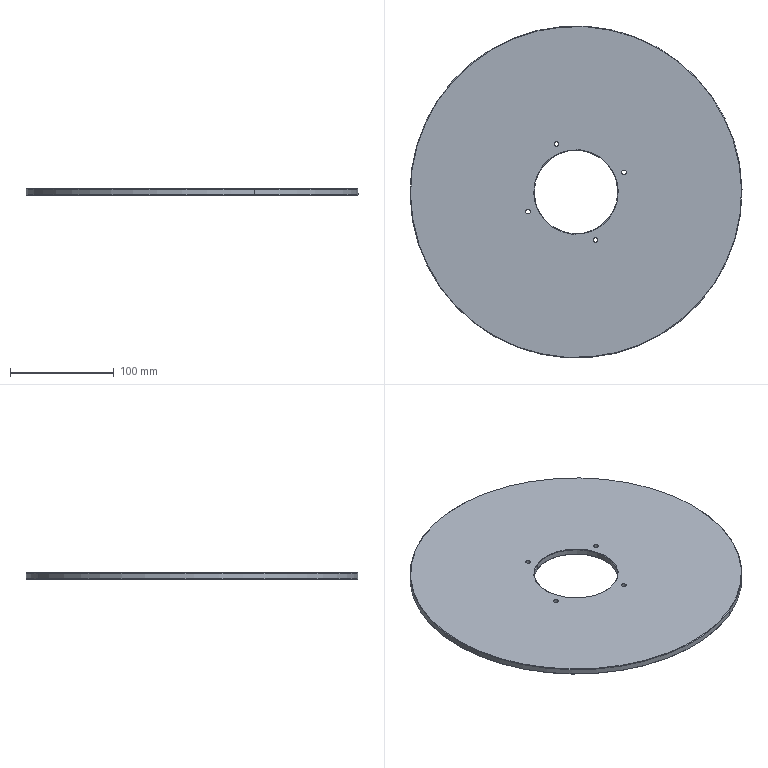Component | SolidWorks | 8TC-A17001-20-05Baffle2-1 | 1 solid | 30 faces | box 320 x 320 x 6 mm | volume 451128 mm3 | cone 16 | cylinder 12 | plane 2 | commonest cylinder face diameters 4.5 x8 80.5 x2 320 x2 | material Tempered Glass
STEP:
#1=COLOUR_RGB('',0.7922,0.8196,0.9333);
#2=FILL_AREA_STYLE_COLOUR('',#1);
#3=FILL_AREA_STYLE('',(#2));
#4=SURFACE_STYLE_FILL_AREA(#3);
#5=SURFACE_SIDE_STYLE('',(#4));
#6=SURFACE_STYLE_USAGE(.BOTH.,#5);
#7=PRESENTATION_STYLE_ASSIGNMENT((#6));
#8=CARTESIAN_POINT('',(26.486,13.716,9.39));
#9=VERTEX_POINT('',#8);
#10=CARTESIAN_POINT('',(31.233,2.089,9.39));
#11=VERTEX_POINT('',#10);
#12=CARTESIAN_POINT('',(28.859,7.902,9.39));
#13=DIRECTION('',(0.,-0.,1.));
#14=DIRECTION('',(-0.378,0.9258,0.));
#15=AXIS2_PLACEMENT_3D('',#12,#13,#14);
#16=CIRCLE('',#15,6.28);
#17=EDGE_CURVE('',#9,#11,#16,.T.);
#18=ORIENTED_EDGE('',*,*,#17,.F.);
#19=CARTESIAN_POINT('',(26.478,13.734,9.37));
#20=VERTEX_POINT('',#19);
#21=CARTESIAN_POINT('',(26.486,13.716,9.39));
#22=DIRECTION('',(-0.2673,0.6546,-0.7071));
#23=VECTOR('',#22,39.37);
#24=LINE('',#21,#23);
#25=EDGE_CURVE('',#9,#20,#24,.T.);
#26=ORIENTED_EDGE('',*,*,#25,.T.);
#27=CARTESIAN_POINT('',(31.241,2.071,9.37));
#28=VERTEX_POINT('',#27);
#29=CARTESIAN_POINT('',(28.859,7.902,9.37));
#30=DIRECTION('',(-0.,0.,-1.));
#31=DIRECTION('',(-0.378,0.9258,0.));
#32=AXIS2_PLACEMENT_3D('',#29,#30,#31);
#33=CIRCLE('',#32,6.299);
#34=EDGE_CURVE('',#28,#20,#33,.T.);
#35=ORIENTED_EDGE('',*,*,#34,.F.);
#36=CARTESIAN_POINT('',(31.233,2.089,9.39));
#37=DIRECTION('',(0.2673,-0.6546,-0.7071));
#38=VECTOR('',#37,39.37);
#39=LINE('',#36,#38);
#40=EDGE_CURVE('',#11,#28,#39,.T.);
#41=ORIENTED_EDGE('',*,*,#40,.F.);
#42=EDGE_LOOP('',(#18,#26,#35,#41));
#43=FACE_OUTER_BOUND('',#42,.T.);
#44=CARTESIAN_POINT('',(28.859,7.902,9.39));
#45=DIRECTION('',(-0.,0.,-1.));
#46=DIRECTION('',(0.378,-0.9258,-0.));
#47=AXIS2_PLACEMENT_3D('',#44,#45,#46);
#48=CONICAL_SURFACE('',#47,6.28,0.7854);
#49=ADVANCED_FACE('',(#43),#48,.T.);
#50=CARTESIAN_POINT('',(31.233,2.089,9.154));
#51=VERTEX_POINT('',#50);
#52=CARTESIAN_POINT('',(26.486,13.716,9.154));
#53=VERTEX_POINT('',#52);
#54=CARTESIAN_POINT('',(28.859,7.902,9.154));
#55=DIRECTION('',(-0.,0.,-1.));
#56=DIRECTION('',(-0.378,0.9258,0.));
#57=AXIS2_PLACEMENT_3D('',#54,#55,#56);
#58=CIRCLE('',#57,6.28);
#59=EDGE_CURVE('',#51,#53,#58,.T.);
#60=ORIENTED_EDGE('',*,*,#59,.F.);
#61=CARTESIAN_POINT('',(31.241,2.071,9.173));
#62=VERTEX_POINT('',#61);
#63=CARTESIAN_POINT('',(31.241,2.071,9.173));
#64=DIRECTION('',(0.2673,-0.6546,0.7071));
#65=VECTOR('',#64,39.37);
#66=LINE('',#63,#65);
#67=EDGE_CURVE('',#51,#62,#66,.T.);
#68=ORIENTED_EDGE('',*,*,#67,.T.);
#69=CARTESIAN_POINT('',(26.478,13.734,9.173));
#70=VERTEX_POINT('',#69);
#71=CARTESIAN_POINT('',(28.859,7.902,9.173));
#72=DIRECTION('',(0.,-0.,1.));
#73=DIRECTION('',(-0.378,0.9258,0.));
#74=AXIS2_PLACEMENT_3D('',#71,#72,#73);
#75=CIRCLE('',#74,6.299);
#76=EDGE_CURVE('',#70,#62,#75,.T.);
#77=ORIENTED_EDGE('',*,*,#76,.F.);
#78=CARTESIAN_POINT('',(26.478,13.734,9.173));
#79=DIRECTION('',(-0.2673,0.6546,0.7071));
#80=VECTOR('',#79,39.37);
#81=LINE('',#78,#80);
#82=EDGE_CURVE('',#53,#70,#81,.T.);
#83=ORIENTED_EDGE('',*,*,#82,.F.);
#84=EDGE_LOOP('',(#60,#68,#77,#83));
#85=FACE_OUTER_BOUND('',#84,.T.);
#86=CARTESIAN_POINT('',(28.859,7.902,9.173));
#87=DIRECTION('',(0.,-0.,1.));
#88=DIRECTION('',(-0.378,0.9258,0.));
#89=AXIS2_PLACEMENT_3D('',#86,#87,#88);
#90=CONICAL_SURFACE('',#89,6.299,0.7854);
#91=ADVANCED_FACE('',(#85),#90,.T.);
#92=CARTESIAN_POINT('',(29.458,6.435,9.37));
#93=VERTEX_POINT('',#92);
#94=CARTESIAN_POINT('',(28.26,9.369,9.37));
#95=VERTEX_POINT('',#94);
#96=CARTESIAN_POINT('',(28.859,7.902,9.37));
#97=DIRECTION('',(0.,-0.,1.));
#98=DIRECTION('',(-0.378,0.9258,0.));
#99=AXIS2_PLACEMENT_3D('',#96,#97,#98);
#100=CIRCLE('',#99,1.585);
#101=EDGE_CURVE('',#93,#95,#100,.T.);
#102=ORIENTED_EDGE('',*,*,#101,.F.);
#103=CARTESIAN_POINT('',(29.466,6.417,9.39));
#104=VERTEX_POINT('',#103);
#105=CARTESIAN_POINT('',(29.458,6.435,9.37));
#106=DIRECTION('',(0.2673,-0.6546,0.7071));
#107=VECTOR('',#106,39.37);
#108=LINE('',#105,#107);
#109=EDGE_CURVE('',#93,#104,#108,.T.);
#110=ORIENTED_EDGE('',*,*,#109,.T.);
#111=CARTESIAN_POINT('',(28.253,9.388,9.39));
#112=VERTEX_POINT('',#111);
#113=CARTESIAN_POINT('',(28.859,7.902,9.39));
#114=DIRECTION('',(-0.,0.,-1.));
#115=DIRECTION('',(-0.378,0.9258,0.));
#116=AXIS2_PLACEMENT_3D('',#113,#114,#115);
#117=CIRCLE('',#116,1.604);
#118=EDGE_CURVE('',#112,#104,#117,.T.);
#119=ORIENTED_EDGE('',*,*,#118,.F.);
#120=CARTESIAN_POINT('',(28.26,9.369,9.37));
#121=DIRECTION('',(-0.2673,0.6546,0.7071));
#122=VECTOR('',#121,39.37);
#123=LINE('',#120,#122);
#124=EDGE_CURVE('',#95,#112,#123,.T.);
#125=ORIENTED_EDGE('',*,*,#124,.F.);
#126=EDGE_LOOP('',(#102,#110,#119,#125));
#127=FACE_OUTER_BOUND('',#126,.T.);
#128=CARTESIAN_POINT('',(28.859,7.902,9.37));
#129=DIRECTION('',(0.,-0.,1.));
#130=DIRECTION('',(-0.378,0.9258,0.));
#131=AXIS2_PLACEMENT_3D('',#128,#129,#130);
#132=CONICAL_SURFACE('',#131,1.585,0.7854);
#133=ADVANCED_FACE('',(#127),#132,.F.);
#134=CARTESIAN_POINT('',(28.26,9.369,9.173));
#135=VERTEX_POINT('',#134);
#136=CARTESIAN_POINT('',(29.458,6.435,9.173));
#137=VERTEX_POINT('',#136);
#138=CARTESIAN_POINT('',(28.859,7.902,9.173));
#139=DIRECTION('',(-0.,0.,-1.));
#140=DIRECTION('',(-0.378,0.9258,0.));
#141=AXIS2_PLACEMENT_3D('',#138,#139,#140);
#142=CIRCLE('',#141,1.585);
#143=EDGE_CURVE('',#135,#137,#142,.T.);
#144=ORIENTED_EDGE('',*,*,#143,.F.);
#145=CARTESIAN_POINT('',(28.253,9.388,9.154));
#146=VERTEX_POINT('',#145);
#147=CARTESIAN_POINT('',(28.253,9.388,9.154));
#148=DIRECTION('',(-0.2673,0.6546,-0.7071));
#149=VECTOR('',#148,39.37);
#150=LINE('',#147,#149);
#151=EDGE_CURVE('',#135,#146,#150,.T.);
#152=ORIENTED_EDGE('',*,*,#151,.T.);
#153=CARTESIAN_POINT('',(29.466,6.417,9.154));
#154=VERTEX_POINT('',#153);
#155=CARTESIAN_POINT('',(28.859,7.902,9.154));
#156=DIRECTION('',(0.,-0.,1.));
#157=DIRECTION('',(-0.378,0.9258,0.));
#158=AXIS2_PLACEMENT_3D('',#155,#156,#157);
#159=CIRCLE('',#158,1.604);
#160=EDGE_CURVE('',#154,#146,#159,.T.);
#161=ORIENTED_EDGE('',*,*,#160,.F.);
#162=CARTESIAN_POINT('',(29.466,6.417,9.154));
#163=DIRECTION('',(0.2673,-0.6546,-0.7071));
#164=VECTOR('',#163,39.37);
#165=LINE('',#162,#164);
#166=EDGE_CURVE('',#137,#154,#165,.T.);
#167=ORIENTED_EDGE('',*,*,#166,.F.);
#168=EDGE_LOOP('',(#144,#152,#161,#167));
#169=FACE_OUTER_BOUND('',#168,.T.);
#170=CARTESIAN_POINT('',(28.859,7.902,9.154));
#171=DIRECTION('',(-0.,0.,-1.));
#172=DIRECTION('',(0.378,-0.9258,0.));
#173=AXIS2_PLACEMENT_3D('',#170,#171,#172);
#174=CONICAL_SURFACE('',#173,1.604,0.7854);
#175=ADVANCED_FACE('',(#169),#174,.F.);
#176=CARTESIAN_POINT('',(27.003,7.24,9.241));
#177=VERTEX_POINT('',#176);
#178=CARTESIAN_POINT('',(27.07,7.076,9.241));
#179=VERTEX_POINT('',#178);
#180=CARTESIAN_POINT('',(27.037,7.158,9.241));
#181=DIRECTION('',(-0.,0.,-1.));
#182=DIRECTION('',(0.378,-0.9258,0.));
#183=AXIS2_PLACEMENT_3D('',#180,#181,#182);
#184=CIRCLE('',#183,0.08858);
#185=EDGE_CURVE('',#177,#179,#184,.T.);
#186=ORIENTED_EDGE('',*,*,#185,.F.);
#187=CARTESIAN_POINT('',(26.97,7.322,9.154));
#188=VERTEX_POINT('',#187);
#189=CARTESIAN_POINT('',(26.97,7.322,9.154));
#190=DIRECTION('',(-0.2673,0.6546,-0.7071));
#191=VECTOR('',#190,39.37);
#192=LINE('',#189,#191);
#193=EDGE_CURVE('',#177,#188,#192,.T.);
#194=ORIENTED_EDGE('',*,*,#193,.T.);
#195=CARTESIAN_POINT('',(27.104,6.995,9.154));
#196=VERTEX_POINT('',#195);
#197=CARTESIAN_POINT('',(27.037,7.158,9.154));
#198=DIRECTION('',(-0.,0.,-1.));
#199=DIRECTION('',(0.378,-0.9258,0.));
#200=AXIS2_PLACEMENT_3D('',#197,#198,#199);
#201=CIRCLE('',#200,0.1764);
#202=EDGE_CURVE('',#188,#196,#201,.T.);
#203=ORIENTED_EDGE('',*,*,#202,.T.);
#204=CARTESIAN_POINT('',(27.104,6.995,9.154));
#205=DIRECTION('',(0.2673,-0.6546,-0.7071));
#206=VECTOR('',#205,39.37);
#207=LINE('',#204,#206);
#208=EDGE_CURVE('',#179,#196,#207,.T.);
#209=ORIENTED_EDGE('',*,*,#208,.F.);
#210=EDGE_LOOP('',(#186,#194,#203,#209));
#211=FACE_OUTER_BOUND('',#210,.T.);
#212=CARTESIAN_POINT('',(27.037,7.158,9.154));
#213=DIRECTION('',(-0.,0.,-1.));
#214=DIRECTION('',(0.378,-0.9258,0.));
#215=AXIS2_PLACEMENT_3D('',#212,#213,#214);
#216=CONICAL_SURFACE('',#215,0.1764,0.7854);
#217=ADVANCED_FACE('',(#211),#216,.F.);
#218=CARTESIAN_POINT('',(27.003,7.24,9.39));
#219=VERTEX_POINT('',#218);
#220=CARTESIAN_POINT('',(27.07,7.076,9.39));
#221=VERTEX_POINT('',#220);
#222=CARTESIAN_POINT('',(27.037,7.158,9.39));
#223=DIRECTION('',(-0.,0.,-1.));
#224=DIRECTION('',(0.378,-0.9258,0.));
#225=AXIS2_PLACEMENT_3D('',#222,#223,#224);
#226=CIRCLE('',#225,0.08858);
#227=EDGE_CURVE('',#219,#221,#226,.T.);
#228=ORIENTED_EDGE('',*,*,#227,.F.);
#229=CARTESIAN_POINT('',(27.003,7.24,9.154));
#230=DIRECTION('',(-0.,0.,-1.));
#231=VECTOR('',#230,39.37);
#232=LINE('',#229,#231);
#233=EDGE_CURVE('',#219,#177,#232,.T.);
#234=ORIENTED_EDGE('',*,*,#233,.T.);
#235=ORIENTED_EDGE('',*,*,#185,.T.);
#236=CARTESIAN_POINT('',(27.07,7.076,9.154));
#237=DIRECTION('',(-0.,0.,-1.));
#238=VECTOR('',#237,39.37);
#239=LINE('',#236,#238);
#240=EDGE_CURVE('',#221,#179,#239,.T.);
#241=ORIENTED_EDGE('',*,*,#240,.F.);
#242=EDGE_LOOP('',(#228,#234,#235,#241));
#243=FACE_OUTER_BOUND('',#242,.T.);
#244=CARTESIAN_POINT('',(27.037,7.158,9.154));
#245=DIRECTION('',(-0.,0.,-1.));
#246=DIRECTION('',(0.378,-0.9258,0.));
#247=AXIS2_PLACEMENT_3D('',#244,#245,#246);
#248=CYLINDRICAL_SURFACE('',#247,0.08858);
#249=ADVANCED_FACE('',(#243),#248,.F.);
#250=CARTESIAN_POINT('',(29.57,6.162,9.241));
#251=VERTEX_POINT('',#250);
#252=CARTESIAN_POINT('',(29.637,5.998,9.241));
#253=VERTEX_POINT('',#252);
#254=CARTESIAN_POINT('',(29.604,6.08,9.241));
#255=DIRECTION('',(-0.,0.,-1.));
#256=DIRECTION('',(0.378,-0.9258,0.));
#257=AXIS2_PLACEMENT_3D('',#254,#255,#256);
#258=CIRCLE('',#257,0.08858);
#259=EDGE_CURVE('',#251,#253,#258,.T.);
#260=ORIENTED_EDGE('',*,*,#259,.F.);
#261=CARTESIAN_POINT('',(29.537,6.243,9.154));
#262=VERTEX_POINT('',#261);
#263=CARTESIAN_POINT('',(29.537,6.243,9.154));
#264=DIRECTION('',(-0.2673,0.6546,-0.7071));
#265=VECTOR('',#264,39.37);
#266=LINE('',#263,#265);
#267=EDGE_CURVE('',#251,#262,#266,.T.);
#268=ORIENTED_EDGE('',*,*,#267,.T.);
#269=CARTESIAN_POINT('',(29.67,5.917,9.154));
#270=VERTEX_POINT('',#269);
#271=CARTESIAN_POINT('',(29.604,6.08,9.154));
#272=DIRECTION('',(-0.,0.,-1.));
#273=DIRECTION('',(0.378,-0.9258,0.));
#274=AXIS2_PLACEMENT_3D('',#271,#272,#273);
#275=CIRCLE('',#274,0.1764);
#276=EDGE_CURVE('',#262,#270,#275,.T.);
#277=ORIENTED_EDGE('',*,*,#276,.T.);
#278=CARTESIAN_POINT('',(29.67,5.917,9.154));
#279=DIRECTION('',(0.2673,-0.6546,-0.7071));
#280=VECTOR('',#279,39.37);
#281=LINE('',#278,#280);
#282=EDGE_CURVE('',#253,#270,#281,.T.);
#283=ORIENTED_EDGE('',*,*,#282,.F.);
#284=EDGE_LOOP('',(#260,#268,#277,#283));
#285=FACE_OUTER_BOUND('',#284,.T.);
#286=CARTESIAN_POINT('',(29.604,6.08,9.154));
#287=DIRECTION('',(-0.,0.,-1.));
#288=DIRECTION('',(0.378,-0.9258,0.));
#289=AXIS2_PLACEMENT_3D('',#286,#287,#288);
#290=CONICAL_SURFACE('',#289,0.1764,0.7854);
#291=ADVANCED_FACE('',(#285),#290,.F.);
#292=CARTESIAN_POINT('',(29.57,6.162,9.39));
#293=VERTEX_POINT('',#292);
#294=CARTESIAN_POINT('',(29.637,5.998,9.39));
#295=VERTEX_POINT('',#294);
#296=CARTESIAN_POINT('',(29.604,6.08,9.39));
#297=DIRECTION('',(-0.,0.,-1.));
#298=DIRECTION('',(0.378,-0.9258,0.));
#299=AXIS2_PLACEMENT_3D('',#296,#297,#298);
#300=CIRCLE('',#299,0.08858);
#301=EDGE_CURVE('',#293,#295,#300,.T.);
#302=ORIENTED_EDGE('',*,*,#301,.F.);
#303=CARTESIAN_POINT('',(29.57,6.162,9.154));
#304=DIRECTION('',(-0.,0.,-1.));
#305=VECTOR('',#304,39.37);
#306=LINE('',#303,#305);
#307=EDGE_CURVE('',#293,#251,#306,.T.);
#308=ORIENTED_EDGE('',*,*,#307,.T.);
#309=ORIENTED_EDGE('',*,*,#259,.T.);
#310=CARTESIAN_POINT('',(29.637,5.998,9.154));
#311=DIRECTION('',(-0.,0.,-1.));
#312=VECTOR('',#311,39.37);
#313=LINE('',#310,#312);
#314=EDGE_CURVE('',#295,#253,#313,.T.);
#315=ORIENTED_EDGE('',*,*,#314,.F.);
#316=EDGE_LOOP('',(#302,#308,#309,#315));
#317=FACE_OUTER_BOUND('',#316,.T.);
#318=CARTESIAN_POINT('',(29.604,6.08,9.154));
#319=DIRECTION('',(-0.,0.,-1.));
#320=DIRECTION('',(0.378,-0.9258,0.));
#321=AXIS2_PLACEMENT_3D('',#318,#319,#320);
#322=CYLINDRICAL_SURFACE('',#321,0.08858);
#323=ADVANCED_FACE('',(#317),#322,.F.);
#324=CARTESIAN_POINT('',(28.082,9.807,9.241));
#325=VERTEX_POINT('',#324);
#326=CARTESIAN_POINT('',(28.149,9.643,9.241));
#327=VERTEX_POINT('',#326);
#328=CARTESIAN_POINT('',(28.115,9.725,9.241));
#329=DIRECTION('',(-0.,0.,-1.));
#330=DIRECTION('',(0.378,-0.9258,0.));
#331=AXIS2_PLACEMENT_3D('',#328,#329,#330);
#332=CIRCLE('',#331,0.08858);
#333=EDGE_CURVE('',#325,#327,#332,.T.);
#334=ORIENTED_EDGE('',*,*,#333,.F.);
#335=CARTESIAN_POINT('',(28.049,9.888,9.154));
#336=VERTEX_POINT('',#335);
#337=CARTESIAN_POINT('',(28.049,9.888,9.154));
#338=DIRECTION('',(-0.2673,0.6546,-0.7071));
#339=VECTOR('',#338,39.37);
#340=LINE('',#337,#339);
#341=EDGE_CURVE('',#325,#336,#340,.T.);
#342=ORIENTED_EDGE('',*,*,#341,.T.);
#343=CARTESIAN_POINT('',(28.182,9.562,9.154));
#344=VERTEX_POINT('',#343);
#345=CARTESIAN_POINT('',(28.115,9.725,9.154));
#346=DIRECTION('',(-0.,0.,-1.));
#347=DIRECTION('',(0.378,-0.9258,0.));
#348=AXIS2_PLACEMENT_3D('',#345,#346,#347);
#349=CIRCLE('',#348,0.1764);
#350=EDGE_CURVE('',#336,#344,#349,.T.);
#351=ORIENTED_EDGE('',*,*,#350,.T.);
#352=CARTESIAN_POINT('',(28.182,9.562,9.154));
#353=DIRECTION('',(0.2673,-0.6546,-0.7071));
#354=VECTOR('',#353,39.37);
#355=LINE('',#352,#354);
#356=EDGE_CURVE('',#327,#344,#355,.T.);
#357=ORIENTED_EDGE('',*,*,#356,.F.);
#358=EDGE_LOOP('',(#334,#342,#351,#357));
#359=FACE_OUTER_BOUND('',#358,.T.);
#360=CARTESIAN_POINT('',(28.115,9.725,9.154));
#361=DIRECTION('',(-0.,0.,-1.));
#362=DIRECTION('',(0.378,-0.9258,0.));
#363=AXIS2_PLACEMENT_3D('',#360,#361,#362);
#364=CONICAL_SURFACE('',#363,0.1764,0.7854);
#365=ADVANCED_FACE('',(#359),#364,.F.);
#366=CARTESIAN_POINT('',(28.082,9.807,9.39));
#367=VERTEX_POINT('',#366);
#368=CARTESIAN_POINT('',(28.149,9.643,9.39));
#369=VERTEX_POINT('',#368);
#370=CARTESIAN_POINT('',(28.115,9.725,9.39));
#371=DIRECTION('',(-0.,0.,-1.));
#372=DIRECTION('',(0.378,-0.9258,0.));
#373=AXIS2_PLACEMENT_3D('',#370,#371,#372);
#374=CIRCLE('',#373,0.08858);
#375=EDGE_CURVE('',#367,#369,#374,.T.);
#376=ORIENTED_EDGE('',*,*,#375,.F.);
#377=CARTESIAN_POINT('',(28.082,9.807,9.154));
#378=DIRECTION('',(-0.,0.,-1.));
#379=VECTOR('',#378,39.37);
#380=LINE('',#377,#379);
#381=EDGE_CURVE('',#367,#325,#380,.T.);
#382=ORIENTED_EDGE('',*,*,#381,.T.);
#383=ORIENTED_EDGE('',*,*,#333,.T.);
#384=CARTESIAN_POINT('',(28.149,9.643,9.154));
#385=DIRECTION('',(-0.,0.,-1.));
#386=VECTOR('',#385,39.37);
#387=LINE('',#384,#386);
#388=EDGE_CURVE('',#369,#327,#387,.T.);
#389=ORIENTED_EDGE('',*,*,#388,.F.);
#390=EDGE_LOOP('',(#376,#382,#383,#389));
#391=FACE_OUTER_BOUND('',#390,.T.);
#392=CARTESIAN_POINT('',(28.115,9.725,9.154));
#393=DIRECTION('',(-0.,0.,-1.));
#394=DIRECTION('',(0.378,-0.9258,0.));
#395=AXIS2_PLACEMENT_3D('',#392,#393,#394);
#396=CYLINDRICAL_SURFACE('',#395,0.08858);
#397=ADVANCED_FACE('',(#391),#396,.F.);
#398=CARTESIAN_POINT('',(30.648,8.729,9.241));
#399=VERTEX_POINT('',#398);
#400=CARTESIAN_POINT('',(30.715,8.565,9.241));
#401=VERTEX_POINT('',#400);
#402=CARTESIAN_POINT('',(30.682,8.647,9.241));
#403=DIRECTION('',(-0.,0.,-1.));
#404=DIRECTION('',(0.378,-0.9258,0.));
#405=AXIS2_PLACEMENT_3D('',#402,#403,#404);
#406=CIRCLE('',#405,0.08858);
#407=EDGE_CURVE('',#399,#401,#406,.T.);
#408=ORIENTED_EDGE('',*,*,#407,.F.);
#409=CARTESIAN_POINT('',(30.615,8.81,9.154));
#410=VERTEX_POINT('',#409);
#411=CARTESIAN_POINT('',(30.615,8.81,9.154));
#412=DIRECTION('',(-0.2673,0.6546,-0.7071));
#413=VECTOR('',#412,39.37);
#414=LINE('',#411,#413);
#415=EDGE_CURVE('',#399,#410,#414,.T.);
#416=ORIENTED_EDGE('',*,*,#415,.T.);
#417=CARTESIAN_POINT('',(30.749,8.483,9.154));
#418=VERTEX_POINT('',#417);
#419=CARTESIAN_POINT('',(30.682,8.647,9.154));
#420=DIRECTION('',(-0.,0.,-1.));
#421=DIRECTION('',(0.378,-0.9258,0.));
#422=AXIS2_PLACEMENT_3D('',#419,#420,#421);
#423=CIRCLE('',#422,0.1764);
#424=EDGE_CURVE('',#410,#418,#423,.T.);
#425=ORIENTED_EDGE('',*,*,#424,.T.);
#426=CARTESIAN_POINT('',(30.749,8.483,9.154));
#427=DIRECTION('',(0.2673,-0.6546,-0.7071));
#428=VECTOR('',#427,39.37);
#429=LINE('',#426,#428);
#430=EDGE_CURVE('',#401,#418,#429,.T.);
#431=ORIENTED_EDGE('',*,*,#430,.F.);
#432=EDGE_LOOP('',(#408,#416,#425,#431));
#433=FACE_OUTER_BOUND('',#432,.T.);
#434=CARTESIAN_POINT('',(30.682,8.647,9.154));
#435=DIRECTION('',(-0.,0.,-1.));
#436=DIRECTION('',(0.378,-0.9258,0.));
#437=AXIS2_PLACEMENT_3D('',#434,#435,#436);
#438=CONICAL_SURFACE('',#437,0.1764,0.7854);
#439=ADVANCED_FACE('',(#433),#438,.F.);
#440=CARTESIAN_POINT('',(30.648,8.729,9.39));
#441=VERTEX_POINT('',#440);
#442=CARTESIAN_POINT('',(30.715,8.565,9.39));
#443=VERTEX_POINT('',#442);
#444=CARTESIAN_POINT('',(30.682,8.647,9.39));
#445=DIRECTION('',(-0.,0.,-1.));
#446=DIRECTION('',(0.378,-0.9258,0.));
#447=AXIS2_PLACEMENT_3D('',#444,#445,#446);
#448=CIRCLE('',#447,0.08858);
#449=EDGE_CURVE('',#441,#443,#448,.T.);
#450=ORIENTED_EDGE('',*,*,#449,.F.);
#451=CARTESIAN_POINT('',(30.648,8.729,9.154));
#452=DIRECTION('',(-0.,0.,-1.));
#453=VECTOR('',#452,39.37);
#454=LINE('',#451,#453);
#455=EDGE_CURVE('',#441,#399,#454,.T.);
#456=ORIENTED_EDGE('',*,*,#455,.T.);
#457=ORIENTED_EDGE('',*,*,#407,.T.);
#458=CARTESIAN_POINT('',(30.715,8.565,9.154));
#459=DIRECTION('',(-0.,0.,-1.));
#460=VECTOR('',#459,39.37);
#461=LINE('',#458,#460);
#462=EDGE_CURVE('',#443,#401,#461,.T.);
#463=ORIENTED_EDGE('',*,*,#462,.F.);
#464=EDGE_LOOP('',(#450,#456,#457,#463));
#465=FACE_OUTER_BOUND('',#464,.T.);
#466=CARTESIAN_POINT('',(30.682,8.647,9.154));
#467=DIRECTION('',(-0.,0.,-1.));
#468=DIRECTION('',(0.378,-0.9258,0.));
#469=AXIS2_PLACEMENT_3D('',#466,#467,#468);
#470=CYLINDRICAL_SURFACE('',#469,0.08858);
#471=ADVANCED_FACE('',(#465),#470,.F.);
#472=ORIENTED_EDGE('',*,*,#101,.T.);
#473=CARTESIAN_POINT('',(28.26,9.369,9.39));
#474=DIRECTION('',(-0.,0.,-1.));
#475=VECTOR('',#474,39.37);
#476=LINE('',#473,#475);
#477=EDGE_CURVE('',#95,#135,#476,.T.);
#478=ORIENTED_EDGE('',*,*,#477,.T.);
#479=ORIENTED_EDGE('',*,*,#143,.T.);
#480=CARTESIAN_POINT('',(29.458,6.435,9.39));
#481=DIRECTION('',(-0.,0.,-1.));
#482=VECTOR('',#481,39.37);
#483=LINE('',#480,#482);
#484=EDGE_CURVE('',#93,#137,#483,.T.);
#485=ORIENTED_EDGE('',*,*,#484,.F.);
#486=EDGE_LOOP('',(#472,#478,#479,#485));
#487=FACE_OUTER_BOUND('',#486,.T.);
#488=CARTESIAN_POINT('',(28.859,7.902,9.39));
#489=DIRECTION('',(-0.,0.,-1.));
#490=DIRECTION('',(0.378,-0.9258,0.));
#491=AXIS2_PLACEMENT_3D('',#488,#489,#490);
#492=CYLINDRICAL_SURFACE('',#491,1.585);
#493=ADVANCED_FACE('',(#487),#492,.F.);
#494=ORIENTED_EDGE('',*,*,#34,.T.);
#495=CARTESIAN_POINT('',(26.478,13.734,9.39));
#496=DIRECTION('',(-0.,0.,-1.));
#497=VECTOR('',#496,39.37);
#498=LINE('',#495,#497);
#499=EDGE_CURVE('',#20,#70,#498,.T.);
#500=ORIENTED_EDGE('',*,*,#499,.T.);
#501=ORIENTED_EDGE('',*,*,#76,.T.);
#502=CARTESIAN_POINT('',(31.241,2.071,9.39));
#503=DIRECTION('',(-0.,0.,-1.));
#504=VECTOR('',#503,39.37);
#505=LINE('',#502,#504);
#506=EDGE_CURVE('',#28,#62,#505,.T.);
#507=ORIENTED_EDGE('',*,*,#506,.F.);
#508=EDGE_LOOP('',(#494,#500,#501,#507));
#509=FACE_OUTER_BOUND('',#508,.T.);
#510=CARTESIAN_POINT('',(28.859,7.902,9.39));
#511=DIRECTION('',(-0.,0.,-1.));
#512=DIRECTION('',(0.378,-0.9258,-0.));
#513=AXIS2_PLACEMENT_3D('',#510,#511,#512);
#514=CYLINDRICAL_SURFACE('',#513,6.299);
#515=ADVANCED_FACE('',(#509),#514,.T.);
#516=ORIENTED_EDGE('',*,*,#118,.T.);
#517=CARTESIAN_POINT('',(28.859,7.902,9.39));
#518=DIRECTION('',(-0.,0.,-1.));
#519=DIRECTION('',(-0.378,0.9258,0.));
#520=AXIS2_PLACEMENT_3D('',#517,#518,#519);
#521=CIRCLE('',#520,1.604);
#522=EDGE_CURVE('',#104,#112,#521,.T.);
#523=ORIENTED_EDGE('',*,*,#522,.T.);
#524=EDGE_LOOP('',(#516,#523));
#525=FACE_BOUND('',#524,.T.);
#526=CARTESIAN_POINT('',(28.859,7.902,9.39));
#527=DIRECTION('',(0.,-0.,1.));
#528=DIRECTION('',(-0.378,0.9258,0.));
#529=AXIS2_PLACEMENT_3D('',#526,#527,#528);
#530=CIRCLE('',#529,6.28);
#531=EDGE_CURVE('',#11,#9,#530,.T.);
#532=ORIENTED_EDGE('',*,*,#531,.T.);
#533=ORIENTED_EDGE('',*,*,#17,.T.);
#534=EDGE_LOOP('',(#532,#533));
#535=FACE_OUTER_BOUND('',#534,.T.);
#536=CARTESIAN_POINT('',(27.037,7.158,9.39));
#537=DIRECTION('',(-0.,0.,-1.));
#538=DIRECTION('',(0.378,-0.9258,0.));
#539=AXIS2_PLACEMENT_3D('',#536,#537,#538);
#540=CIRCLE('',#539,0.08858);
#541=EDGE_CURVE('',#221,#219,#540,.T.);
#542=ORIENTED_EDGE('',*,*,#541,.T.);
#543=ORIENTED_EDGE('',*,*,#227,.T.);
#544=EDGE_LOOP('',(#542,#543));
#545=FACE_BOUND('',#544,.T.);
#546=CARTESIAN_POINT('',(29.604,6.08,9.39));
#547=DIRECTION('',(-0.,0.,-1.));
#548=DIRECTION('',(0.378,-0.9258,0.));
#549=AXIS2_PLACEMENT_3D('',#546,#547,#548);
#550=CIRCLE('',#549,0.08858);
#551=EDGE_CURVE('',#295,#293,#550,.T.);
#552=ORIENTED_EDGE('',*,*,#551,.T.);
#553=ORIENTED_EDGE('',*,*,#301,.T.);
#554=EDGE_LOOP('',(#552,#553));
#555=FACE_BOUND('',#554,.T.);
#556=CARTESIAN_POINT('',(28.115,9.725,9.39));
#557=DIRECTION('',(-0.,0.,-1.));
#558=DIRECTION('',(0.378,-0.9258,0.));
#559=AXIS2_PLACEMENT_3D('',#556,#557,#558);
#560=CIRCLE('',#559,0.08858);
#561=EDGE_CURVE('',#369,#367,#560,.T.);
#562=ORIENTED_EDGE('',*,*,#561,.T.);
#563=ORIENTED_EDGE('',*,*,#375,.T.);
#564=EDGE_LOOP('',(#562,#563));
#565=FACE_BOUND('',#564,.T.);
#566=CARTESIAN_POINT('',(30.682,8.647,9.39));
#567=DIRECTION('',(-0.,0.,-1.));
#568=DIRECTION('',(0.378,-0.9258,0.));
#569=AXIS2_PLACEMENT_3D('',#566,#567,#568);
#570=CIRCLE('',#569,0.08858);
#571=EDGE_CURVE('',#443,#441,#570,.T.);
#572=ORIENTED_EDGE('',*,*,#571,.T.);
#573=ORIENTED_EDGE('',*,*,#449,.T.);
#574=EDGE_LOOP('',(#572,#573));
#575=FACE_BOUND('',#574,.T.);
#576=CARTESIAN_POINT('',(28.859,7.902,9.39));
#577=DIRECTION('',(0.,-0.,1.));
#578=DIRECTION('',(-0.378,0.9258,0.));
#579=AXIS2_PLACEMENT_3D('',#576,#577,#578);
#580=PLANE('',#579);
#581=ADVANCED_FACE('',(#525,#535,#545,#555,#565,#575),#580,.T.);
#582=ORIENTED_EDGE('',*,*,#160,.T.);
#583=CARTESIAN_POINT('',(28.859,7.902,9.154));
#584=DIRECTION('',(0.,-0.,1.));
#585=DIRECTION('',(-0.378,0.9258,0.));
#586=AXIS2_PLACEMENT_3D('',#583,#584,#585);
#587=CIRCLE('',#586,1.604);
#588=EDGE_CURVE('',#146,#154,#587,.T.);
#589=ORIENTED_EDGE('',*,*,#588,.T.);
#590=EDGE_LOOP('',(#582,#589));
#591=FACE_BOUND('',#590,.T.);
#592=CARTESIAN_POINT('',(28.859,7.902,9.154));
#593=DIRECTION('',(-0.,0.,-1.));
#594=DIRECTION('',(-0.378,0.9258,0.));
#595=AXIS2_PLACEMENT_3D('',#592,#593,#594);
#596=CIRCLE('',#595,6.28);
#597=EDGE_CURVE('',#53,#51,#596,.T.);
#598=ORIENTED_EDGE('',*,*,#597,.T.);
#599=ORIENTED_EDGE('',*,*,#59,.T.);
#600=EDGE_LOOP('',(#598,#599));
#601=FACE_OUTER_BOUND('',#600,.T.);
#602=CARTESIAN_POINT('',(27.037,7.158,9.154));
#603=DIRECTION('',(-0.,0.,-1.));
#604=DIRECTION('',(0.378,-0.9258,0.));
#605=AXIS2_PLACEMENT_3D('',#602,#603,#604);
#606=CIRCLE('',#605,0.1764);
#607=EDGE_CURVE('',#196,#188,#606,.T.);
#608=ORIENTED_EDGE('',*,*,#607,.F.);
#609=ORIENTED_EDGE('',*,*,#202,.F.);
#610=EDGE_LOOP('',(#608,#609));
#611=FACE_BOUND('',#610,.T.);
#612=CARTESIAN_POINT('',(29.604,6.08,9.154));
#613=DIRECTION('',(-0.,0.,-1.));
#614=DIRECTION('',(0.378,-0.9258,0.));
#615=AXIS2_PLACEMENT_3D('',#612,#613,#614);
#616=CIRCLE('',#615,0.1764);
#617=EDGE_CURVE('',#270,#262,#616,.T.);
#618=ORIENTED_EDGE('',*,*,#617,.F.);
#619=ORIENTED_EDGE('',*,*,#276,.F.);
#620=EDGE_LOOP('',(#618,#619));
#621=FACE_BOUND('',#620,.T.);
#622=CARTESIAN_POINT('',(28.115,9.725,9.154));
#623=DIRECTION('',(-0.,0.,-1.));
#624=DIRECTION('',(0.378,-0.9258,0.));
#625=AXIS2_PLACEMENT_3D('',#622,#623,#624);
#626=CIRCLE('',#625,0.1764);
#627=EDGE_CURVE('',#344,#336,#626,.T.);
#628=ORIENTED_EDGE('',*,*,#627,.F.);
#629=ORIENTED_EDGE('',*,*,#350,.F.);
#630=EDGE_LOOP('',(#628,#629));
#631=FACE_BOUND('',#630,.T.);
#632=CARTESIAN_POINT('',(30.682,8.647,9.154));
#633=DIRECTION('',(-0.,0.,-1.));
#634=DIRECTION('',(0.378,-0.9258,0.));
#635=AXIS2_PLACEMENT_3D('',#632,#633,#634);
#636=CIRCLE('',#635,0.1764);
#637=EDGE_CURVE('',#418,#410,#636,.T.);
#638=ORIENTED_EDGE('',*,*,#637,.F.);
#639=ORIENTED_EDGE('',*,*,#424,.F.);
#640=EDGE_LOOP('',(#638,#639));
#641=FACE_BOUND('',#640,.T.);
#642=CARTESIAN_POINT('',(28.859,7.902,9.154));
#643=DIRECTION('',(0.,-0.,1.));
#644=DIRECTION('',(-0.378,0.9258,0.));
#645=AXIS2_PLACEMENT_3D('',#642,#643,#644);
#646=PLANE('',#645);
#647=ADVANCED_FACE('',(#591,#601,#611,#621,#631,#641),#646,.F.);
#648=ORIENTED_EDGE('',*,*,#499,.F.);
#649=CARTESIAN_POINT('',(28.859,7.902,9.37));
#650=DIRECTION('',(-0.,0.,-1.));
#651=DIRECTION('',(-0.378,0.9258,0.));
#652=AXIS2_PLACEMENT_3D('',#649,#650,#651);
#653=CIRCLE('',#652,6.299);
#654=EDGE_CURVE('',#20,#28,#653,.T.);
#655=ORIENTED_EDGE('',*,*,#654,.T.);
#656=ORIENTED_EDGE('',*,*,#506,.T.);
#657=CARTESIAN_POINT('',(28.859,7.902,9.173));
#658=DIRECTION('',(0.,-0.,1.));
#659=DIRECTION('',(-0.378,0.9258,0.));
#660=AXIS2_PLACEMENT_3D('',#657,#658,#659);
#661=CIRCLE('',#660,6.299);
#662=EDGE_CURVE('',#62,#70,#661,.T.);
#663=ORIENTED_EDGE('',*,*,#662,.T.);
#664=EDGE_LOOP('',(#648,#655,#656,#663));
#665=FACE_OUTER_BOUND('',#664,.T.);
#666=CARTESIAN_POINT('',(28.859,7.902,9.39));
#667=DIRECTION('',(-0.,0.,-1.));
#668=DIRECTION('',(0.378,-0.9258,-0.));
#669=AXIS2_PLACEMENT_3D('',#666,#667,#668);
#670=CYLINDRICAL_SURFACE('',#669,6.299);
#671=ADVANCED_FACE('',(#665),#670,.T.);
#672=ORIENTED_EDGE('',*,*,#477,.F.);
#673=CARTESIAN_POINT('',(28.859,7.902,9.37));
#674=DIRECTION('',(0.,-0.,1.));
#675=DIRECTION('',(-0.378,0.9258,0.));
#676=AXIS2_PLACEMENT_3D('',#673,#674,#675);
#677=CIRCLE('',#676,1.585);
#678=EDGE_CURVE('',#95,#93,#677,.T.);
#679=ORIENTED_EDGE('',*,*,#678,.T.);
#680=ORIENTED_EDGE('',*,*,#484,.T.);
#681=CARTESIAN_POINT('',(28.859,7.902,9.173));
#682=DIRECTION('',(-0.,0.,-1.));
#683=DIRECTION('',(-0.378,0.9258,0.));
#684=AXIS2_PLACEMENT_3D('',#681,#682,#683);
#685=CIRCLE('',#684,1.585);
#686=EDGE_CURVE('',#137,#135,#685,.T.);
#687=ORIENTED_EDGE('',*,*,#686,.T.);
#688=EDGE_LOOP('',(#672,#679,#680,#687));
#689=FACE_OUTER_BOUND('',#688,.T.);
#690=CARTESIAN_POINT('',(28.859,7.902,9.39));
#691=DIRECTION('',(-0.,0.,-1.));
#692=DIRECTION('',(0.378,-0.9258,0.));
#693=AXIS2_PLACEMENT_3D('',#690,#691,#692);
#694=CYLINDRICAL_SURFACE('',#693,1.585);
#695=ADVANCED_FACE('',(#689),#694,.F.);
#696=ORIENTED_EDGE('',*,*,#455,.F.);
#697=ORIENTED_EDGE('',*,*,#571,.F.);
#698=ORIENTED_EDGE('',*,*,#462,.T.);
#699=CARTESIAN_POINT('',(30.682,8.647,9.241));
#700=DIRECTION('',(-0.,0.,-1.));
#701=DIRECTION('',(0.378,-0.9258,0.));
#702=AXIS2_PLACEMENT_3D('',#699,#700,#701);
#703=CIRCLE('',#702,0.08858);
#704=EDGE_CURVE('',#401,#399,#703,.T.);
#705=ORIENTED_EDGE('',*,*,#704,.T.);
#706=EDGE_LOOP('',(#696,#697,#698,#705));
#707=FACE_OUTER_BOUND('',#706,.T.);
#708=CARTESIAN_POINT('',(30.682,8.647,9.154));
#709=DIRECTION('',(-0.,0.,-1.));
#710=DIRECTION('',(0.378,-0.9258,0.));
#711=AXIS2_PLACEMENT_3D('',#708,#709,#710);
#712=CYLINDRICAL_SURFACE('',#711,0.08858);
#713=ADVANCED_FACE('',(#707),#712,.F.);
#714=ORIENTED_EDGE('',*,*,#415,.F.);
#715=ORIENTED_EDGE('',*,*,#704,.F.);
#716=ORIENTED_EDGE('',*,*,#430,.T.);
#717=ORIENTED_EDGE('',*,*,#637,.T.);
#718=EDGE_LOOP('',(#714,#715,#716,#717));
#719=FACE_OUTER_BOUND('',#718,.T.);
#720=CARTESIAN_POINT('',(30.682,8.647,9.154));
#721=DIRECTION('',(-0.,0.,-1.));
#722=DIRECTION('',(0.378,-0.9258,0.));
#723=AXIS2_PLACEMENT_3D('',#720,#721,#722);
#724=CONICAL_SURFACE('',#723,0.1764,0.7854);
#725=ADVANCED_FACE('',(#719),#724,.F.);
#726=ORIENTED_EDGE('',*,*,#381,.F.);
#727=ORIENTED_EDGE('',*,*,#561,.F.);
#728=ORIENTED_EDGE('',*,*,#388,.T.);
#729=CARTESIAN_POINT('',(28.115,9.725,9.241));
#730=DIRECTION('',(-0.,0.,-1.));
#731=DIRECTION('',(0.378,-0.9258,0.));
#732=AXIS2_PLACEMENT_3D('',#729,#730,#731);
#733=CIRCLE('',#732,0.08858);
#734=EDGE_CURVE('',#327,#325,#733,.T.);
#735=ORIENTED_EDGE('',*,*,#734,.T.);
#736=EDGE_LOOP('',(#726,#727,#728,#735));
#737=FACE_OUTER_BOUND('',#736,.T.);
#738=CARTESIAN_POINT('',(28.115,9.725,9.154));
#739=DIRECTION('',(-0.,0.,-1.));
#740=DIRECTION('',(0.378,-0.9258,0.));
#741=AXIS2_PLACEMENT_3D('',#738,#739,#740);
#742=CYLINDRICAL_SURFACE('',#741,0.08858);
#743=ADVANCED_FACE('',(#737),#742,.F.);
#744=ORIENTED_EDGE('',*,*,#341,.F.);
#745=ORIENTED_EDGE('',*,*,#734,.F.);
#746=ORIENTED_EDGE('',*,*,#356,.T.);
#747=ORIENTED_EDGE('',*,*,#627,.T.);
#748=EDGE_LOOP('',(#744,#745,#746,#747));
#749=FACE_OUTER_BOUND('',#748,.T.);
#750=CARTESIAN_POINT('',(28.115,9.725,9.154));
#751=DIRECTION('',(-0.,0.,-1.));
#752=DIRECTION('',(0.378,-0.9258,0.));
#753=AXIS2_PLACEMENT_3D('',#750,#751,#752);
#754=CONICAL_SURFACE('',#753,0.1764,0.7854);
#755=ADVANCED_FACE('',(#749),#754,.F.);
#756=ORIENTED_EDGE('',*,*,#307,.F.);
#757=ORIENTED_EDGE('',*,*,#551,.F.);
#758=ORIENTED_EDGE('',*,*,#314,.T.);
#759=CARTESIAN_POINT('',(29.604,6.08,9.241));
#760=DIRECTION('',(-0.,0.,-1.));
#761=DIRECTION('',(0.378,-0.9258,0.));
#762=AXIS2_PLACEMENT_3D('',#759,#760,#761);
#763=CIRCLE('',#762,0.08858);
#764=EDGE_CURVE('',#253,#251,#763,.T.);
#765=ORIENTED_EDGE('',*,*,#764,.T.);
#766=EDGE_LOOP('',(#756,#757,#758,#765));
#767=FACE_OUTER_BOUND('',#766,.T.);
#768=CARTESIAN_POINT('',(29.604,6.08,9.154));
#769=DIRECTION('',(-0.,0.,-1.));
#770=DIRECTION('',(0.378,-0.9258,0.));
#771=AXIS2_PLACEMENT_3D('',#768,#769,#770);
#772=CYLINDRICAL_SURFACE('',#771,0.08858);
#773=ADVANCED_FACE('',(#767),#772,.F.);
#774=ORIENTED_EDGE('',*,*,#267,.F.);
#775=ORIENTED_EDGE('',*,*,#764,.F.);
#776=ORIENTED_EDGE('',*,*,#282,.T.);
#777=ORIENTED_EDGE('',*,*,#617,.T.);
#778=EDGE_LOOP('',(#774,#775,#776,#777));
#779=FACE_OUTER_BOUND('',#778,.T.);
#780=CARTESIAN_POINT('',(29.604,6.08,9.154));
#781=DIRECTION('',(-0.,0.,-1.));
#782=DIRECTION('',(0.378,-0.9258,0.));
#783=AXIS2_PLACEMENT_3D('',#780,#781,#782);
#784=CONICAL_SURFACE('',#783,0.1764,0.7854);
#785=ADVANCED_FACE('',(#779),#784,.F.);
#786=ORIENTED_EDGE('',*,*,#233,.F.);
#787=ORIENTED_EDGE('',*,*,#541,.F.);
#788=ORIENTED_EDGE('',*,*,#240,.T.);
#789=CARTESIAN_POINT('',(27.037,7.158,9.241));
#790=DIRECTION('',(-0.,0.,-1.));
#791=DIRECTION('',(0.378,-0.9258,0.));
#792=AXIS2_PLACEMENT_3D('',#789,#790,#791);
#793=CIRCLE('',#792,0.08858);
#794=EDGE_CURVE('',#179,#177,#793,.T.);
#795=ORIENTED_EDGE('',*,*,#794,.T.);
#796=EDGE_LOOP('',(#786,#787,#788,#795));
#797=FACE_OUTER_BOUND('',#796,.T.);
#798=CARTESIAN_POINT('',(27.037,7.158,9.154));
#799=DIRECTION('',(-0.,0.,-1.));
#800=DIRECTION('',(0.378,-0.9258,0.));
#801=AXIS2_PLACEMENT_3D('',#798,#799,#800);
#802=CYLINDRICAL_SURFACE('',#801,0.08858);
#803=ADVANCED_FACE('',(#797),#802,.F.);
#804=ORIENTED_EDGE('',*,*,#193,.F.);
#805=ORIENTED_EDGE('',*,*,#794,.F.);
#806=ORIENTED_EDGE('',*,*,#208,.T.);
#807=ORIENTED_EDGE('',*,*,#607,.T.);
#808=EDGE_LOOP('',(#804,#805,#806,#807));
#809=FACE_OUTER_BOUND('',#808,.T.);
#810=CARTESIAN_POINT('',(27.037,7.158,9.154));
#811=DIRECTION('',(-0.,0.,-1.));
#812=DIRECTION('',(0.378,-0.9258,0.));
#813=AXIS2_PLACEMENT_3D('',#810,#811,#812);
#814=CONICAL_SURFACE('',#813,0.1764,0.7854);
#815=ADVANCED_FACE('',(#809),#814,.F.);
#816=ORIENTED_EDGE('',*,*,#151,.F.);
#817=ORIENTED_EDGE('',*,*,#686,.F.);
#818=ORIENTED_EDGE('',*,*,#166,.T.);
#819=ORIENTED_EDGE('',*,*,#588,.F.);
#820=EDGE_LOOP('',(#816,#817,#818,#819));
#821=FACE_OUTER_BOUND('',#820,.T.);
#822=CARTESIAN_POINT('',(28.859,7.902,9.154));
#823=DIRECTION('',(-0.,0.,-1.));
#824=DIRECTION('',(0.378,-0.9258,0.));
#825=AXIS2_PLACEMENT_3D('',#822,#823,#824);
#826=CONICAL_SURFACE('',#825,1.604,0.7854);
#827=ADVANCED_FACE('',(#821),#826,.F.);
#828=ORIENTED_EDGE('',*,*,#109,.F.);
#829=ORIENTED_EDGE('',*,*,#678,.F.);
#830=ORIENTED_EDGE('',*,*,#124,.T.);
#831=ORIENTED_EDGE('',*,*,#522,.F.);
#832=EDGE_LOOP('',(#828,#829,#830,#831));
#833=FACE_OUTER_BOUND('',#832,.T.);
#834=CARTESIAN_POINT('',(28.859,7.902,9.37));
#835=DIRECTION('',(0.,-0.,1.));
#836=DIRECTION('',(-0.378,0.9258,0.));
#837=AXIS2_PLACEMENT_3D('',#834,#835,#836);
#838=CONICAL_SURFACE('',#837,1.585,0.7854);
#839=ADVANCED_FACE('',(#833),#838,.F.);
#840=ORIENTED_EDGE('',*,*,#67,.F.);
#841=ORIENTED_EDGE('',*,*,#597,.F.);
#842=ORIENTED_EDGE('',*,*,#82,.T.);
#843=ORIENTED_EDGE('',*,*,#662,.F.);
#844=EDGE_LOOP('',(#840,#841,#842,#843));
#845=FACE_OUTER_BOUND('',#844,.T.);
#846=CARTESIAN_POINT('',(28.859,7.902,9.173));
#847=DIRECTION('',(0.,-0.,1.));
#848=DIRECTION('',(-0.378,0.9258,0.));
#849=AXIS2_PLACEMENT_3D('',#846,#847,#848);
#850=CONICAL_SURFACE('',#849,6.299,0.7854);
#851=ADVANCED_FACE('',(#845),#850,.T.);
#852=ORIENTED_EDGE('',*,*,#25,.F.);
#853=ORIENTED_EDGE('',*,*,#531,.F.);
#854=ORIENTED_EDGE('',*,*,#40,.T.);
#855=ORIENTED_EDGE('',*,*,#654,.F.);
#856=EDGE_LOOP('',(#852,#853,#854,#855));
#857=FACE_OUTER_BOUND('',#856,.T.);
#858=CARTESIAN_POINT('',(28.859,7.902,9.39));
#859=DIRECTION('',(-0.,0.,-1.));
#860=DIRECTION('',(0.378,-0.9258,-0.));
#861=AXIS2_PLACEMENT_3D('',#858,#859,#860);
#862=CONICAL_SURFACE('',#861,6.28,0.7854);
#863=ADVANCED_FACE('',(#857),#862,.T.);
#864=CLOSED_SHELL('',(#49,#91,#133,#175,#217,#249,#291,#323,#365,#397,#439,#471,#493,#515,#581,#647,#671,#695,#713,#725,#743,#755,#773,#785,#803,#815,#827,#839,#851,#863));
#865=MANIFOLD_SOLID_BREP('',#864);
#866=STYLED_ITEM('',(#7),#865);
#867=(LENGTH_UNIT()NAMED_UNIT(*)SI_UNIT($,.METRE.));
#868=LENGTH_MEASURE_WITH_UNIT(LENGTH_MEASURE(0.0254),#867);
#869=DIMENSIONAL_EXPONENTS(1.,0.,0.,0.,0.,0.,0.);
#870=(CONVERSION_BASED_UNIT('',#868)LENGTH_UNIT()NAMED_UNIT(#869));
#871=UNCERTAINTY_MEASURE_WITH_UNIT(LENGTH_MEASURE(0.00001),#870,'','');
#872=(NAMED_UNIT(*)PLANE_ANGLE_UNIT()SI_UNIT($,.RADIAN.));
#873=(NAMED_UNIT(*)SI_UNIT($,.STERADIAN.)SOLID_ANGLE_UNIT());
#874=(GEOMETRIC_REPRESENTATION_CONTEXT(3)GLOBAL_UNCERTAINTY_ASSIGNED_CONTEXT((#871))GLOBAL_UNIT_ASSIGNED_CONTEXT((#870,#872,#873))REPRESENTATION_CONTEXT('',''));
#875=MECHANICAL_DESIGN_GEOMETRIC_PRESENTATION_REPRESENTATION('',(#866),#874);
#876=PRESENTATION_LAYER_ASSIGNMENT('','',(#866));
#877=CARTESIAN_POINT('',(0.,0.,0.));
#878=DIRECTION('',(0.,0.,1.));
#879=DIRECTION('',(1.,0.,0.));
#880=AXIS2_PLACEMENT_3D('',#877,#878,#879);
#881=(LENGTH_UNIT()NAMED_UNIT(*)SI_UNIT($,.METRE.));
#882=LENGTH_MEASURE_WITH_UNIT(LENGTH_MEASURE(0.0254),#881);
#883=DIMENSIONAL_EXPONENTS(1.,0.,0.,0.,0.,0.,0.);
#884=(CONVERSION_BASED_UNIT('',#882)LENGTH_UNIT()NAMED_UNIT(#883));
#885=UNCERTAINTY_MEASURE_WITH_UNIT(LENGTH_MEASURE(0.00001),#884,'','');
#886=(NAMED_UNIT(*)PLANE_ANGLE_UNIT()SI_UNIT($,.RADIAN.));
#887=(NAMED_UNIT(*)SI_UNIT($,.STERADIAN.)SOLID_ANGLE_UNIT());
#888=(GEOMETRIC_REPRESENTATION_CONTEXT(3)GLOBAL_UNCERTAINTY_ASSIGNED_CONTEXT((#885))GLOBAL_UNIT_ASSIGNED_CONTEXT((#884,#886,#887))REPRESENTATION_CONTEXT('',''));
#889=ADVANCED_BREP_SHAPE_REPRESENTATION('',(#865,#880),#888);